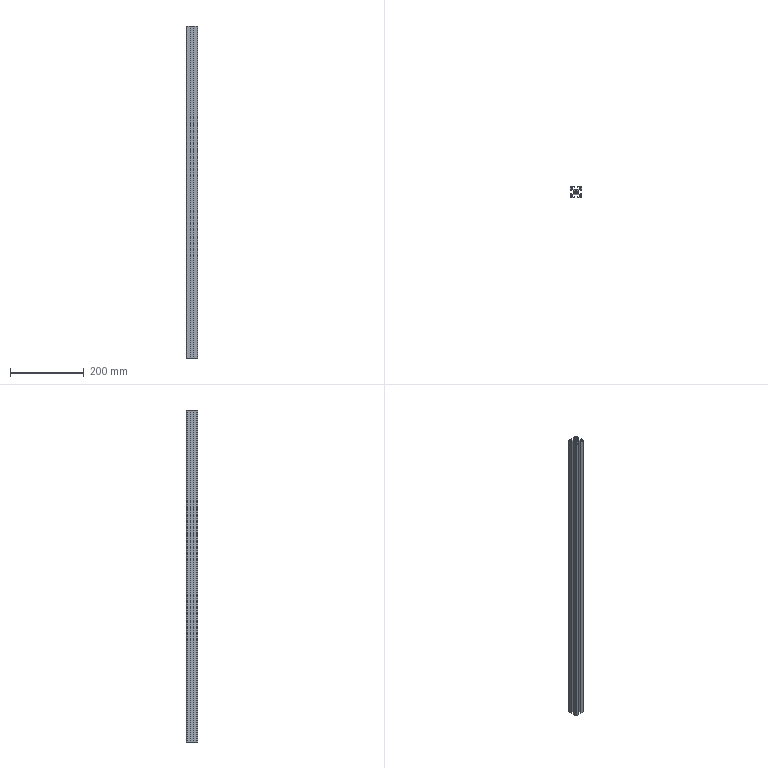Component | SolidWorks | 3030-900-4 | 1 solid | 64 faces | box 30 x 30 x 900 mm | volume 301182 mm3 | plane 46 | cylinder 18 | commonest cylinder face diameters 4.2 x8 0.6 x4 4 x4 6.8 x2
build123d program:
from build123d import *

# Parameters (mm, degrees)
SKETCH1_R           = 2.1
SKETCH1_R_2         = 3.4
BOSS_EXTRUDE1_DEPTH = 900


with BuildPart() as part:
    # Sketch1 → Boss-Extrude1 (new body)
    with BuildSketch(Plane(origin=(0, 0, -100), x_dir=(-1, 0, 0), z_dir=(0, 0, -1))):
        with BuildLine():
            Line((15, 3.8), (15, 13.5))
            ThreePointArc((15, 13.5), (14.823, 14.323), (14.323, 15))
            Line((14.323, 15), (4, 15))
            Line((4, 15), (4, 13))
            Line((4, 13), (8.25, 13))
            Line((8.25, 13), (8.25, 9.664))
            Line((8.25, 9.664), (4.586, 6))
            Line((4.586, 6), (-4.586, 6))
            Line((-4.586, 6), (-8.25, 9.664))
            Line((-8.25, 9.664), (-8.25, 13))
            Line((-8.25, 13), (-4, 13))
            Line((-4, 13), (-4, 15))
            Line((-4, 15), (-14.323, 15))
            ThreePointArc((-14.323, 15), (-14.823, 14.323), (-15, 13.5))
            Line((-15, 13.5), (-15, 3.8))
            ThreePointArc((-15, 3.8), (-14.912, 3.588), (-14.7, 3.5))
            Line((-14.7, 3.5), (-13, 3.5))
            Line((-13, 3.5), (-13, 8.25))
            Line((-13, 8.25), (-9.664, 8.25))
            Line((-9.664, 8.25), (-6, 4.586))
            Line((-6, 4.586), (-6, -4.586))
            Line((-6, -4.586), (-9.664, -8.25))
            Line((-9.664, -8.25), (-13, -8.25))
            Line((-13, -8.25), (-13, -4.5))
            Line((-13, -4.5), (-14.7, -4.5))
            ThreePointArc((-14.7, -4.5), (-14.912, -4.588), (-15, -4.8))
            Line((-15, -4.8), (-15, -13.5))
            ThreePointArc((-15, -13.5), (-14.823, -14.323), (-14.323, -15))
            Line((-14.323, -15), (-4, -15))
            Line((-4, -15), (-4, -13))
            Line((-4, -13), (-8.25, -13))
            Line((-8.25, -13), (-8.25, -9.664))
            Line((-8.25, -9.664), (-4.586, -6))
            Line((-4.586, -6), (4.586, -6))
            Line((4.586, -6), (8.25, -9.664))
            Line((8.25, -9.664), (8.25, -13))
            Line((8.25, -13), (4, -13))
            Line((4, -13), (4, -15))
            Line((4, -15), (14.323, -15))
            ThreePointArc((14.323, -15), (14.823, -14.323), (15, -13.5))
            Line((15, -13.5), (15, -4.8))
            ThreePointArc((15, -4.8), (14.912, -4.588), (14.7, -4.5))
            Line((14.7, -4.5), (13, -4.5))
            Line((13, -4.5), (13, -8.25))
            Line((13, -8.25), (9.664, -8.25))
            Line((9.664, -8.25), (6, -4.586))
            Line((6, -4.586), (6, 4.586))
            Line((6, 4.586), (9.664, 8.25))
            Line((9.664, 8.25), (13, 8.25))
            Line((13, 8.25), (13, 3.5))
            Line((13, 3.5), (14.7, 3.5))
            ThreePointArc((14.7, 3.5), (14.912, 3.588), (15, 3.8))
        make_face()
        with Locations(Location((11.625, 11.625, 0), (0, 0, 180))):
            Circle(SKETCH1_R, mode=Mode.SUBTRACT)
        with Locations(Location((11.625, -11.625, 0), (0, 0, 180))):
            Circle(SKETCH1_R, mode=Mode.SUBTRACT)
        with Locations(Location((0, 0, 0), (0, 0, 180))):
            Circle(SKETCH1_R_2, mode=Mode.SUBTRACT)
        with Locations(Location((-11.625, 11.625, 0), (0, 0, 180))):
            Circle(SKETCH1_R, mode=Mode.SUBTRACT)
        with Locations(Location((-11.625, -11.625, 0), (0, 0, 180))):
            Circle(SKETCH1_R, mode=Mode.SUBTRACT)
    extrude(amount=-BOSS_EXTRUDE1_DEPTH)


solid = part.part

# Placed as in the assembly
solid = solid.moved(Location((-13.047, 637.523, -350), (0, 0, 0)))